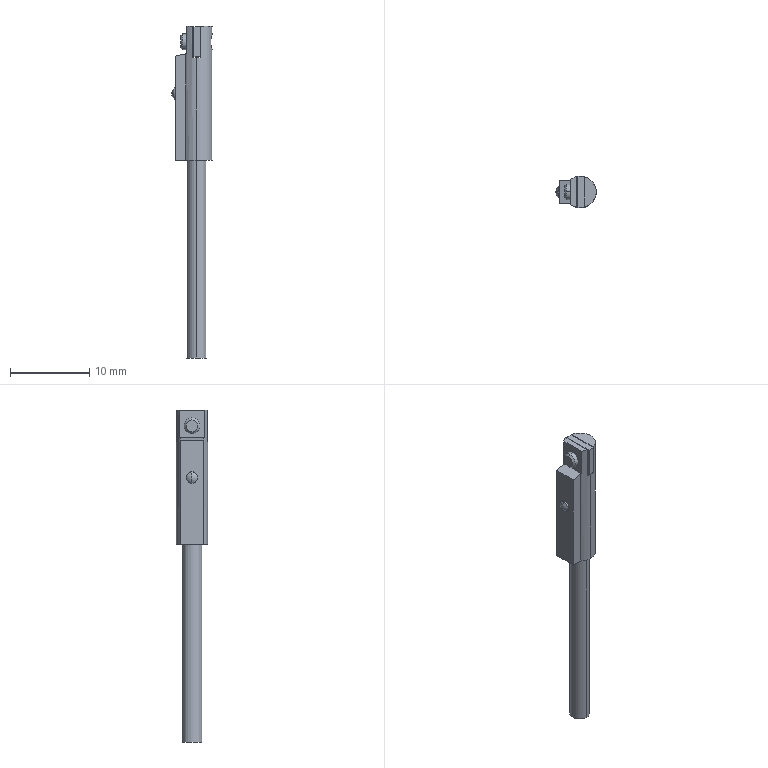Component | SolidWorks | SL010-LeftStreamline-1-1_SL010-SideClampAssembly-DB-1-1_SL010-HLQ8X10SAF(0)+(DS1-H-2)-DB-1-1_SL010-DS1-H-DB-1-1 | 1 solid | 45 faces | box 5.1 x 4 x 42 mm | volume 361 mm3 | plane 22 | cylinder 13 | cone 6 | torus 2 | sphere 2 | commonest cylinder face diameters 2 x4 4 x3 2.5 x2 1.5 x2 1.567 x2
build123d program:
from build123d import *

# Parameters (mm, degrees)
BOSS_EXTRUDE1_DEPTH      = 17
CUT_EXTRUDE1_DEPTH       = 2.5
CUT_EXTRUDE1_DEPTH_BACK  = 2.5
CUT_EXTRUDE2_DEPTH       = 4
CUT_EXTRUDE2_DEPTH_BACK  = 4
SKETCH4_W                = 4
SKETCH4_H                = 1
BOSS_EXTRUDE2_DEPTH      = 2
BOSS_EXTRUDE2_DEPTH_BACK = 2
SKETCH5_W                = 3.8
SKETCH5_H                = 0.8
SKETCH8_W                = 25
SKETCH8_H                = 1.25


with BuildPart() as part:
    # Sketch1 → Boss-Extrude1 (new body)
    with BuildSketch(Plane.XY):
        with BuildLine():
            Line((1.5, 1.323), (1.5, 2.6))
            Line((1.5, 2.6), (-1.5, 2.6))
            Line((-1.5, 2.6), (-1.5, 1.323))
            ThreePointArc((-1.5, 1.323), (0, -2), (1.5, 1.323))
        make_face()
    extrude(amount=BOSS_EXTRUDE1_DEPTH)

    # Sketch2 → Cut-Extrude1 (cut, two sides: drawn at the far end of the back side and taken through both)
    with BuildSketch(Plane(origin=(0, 0, 0), x_dir=(0, 0, -1), z_dir=(1, 0, 0)).offset(-CUT_EXTRUDE1_DEPTH_BACK)):
        Polygon((-17, 2.6), (-17, 1.22), (-13.5, 1.22), (-13.2, 2.6), align=None)
    extrude(amount=CUT_EXTRUDE1_DEPTH + CUT_EXTRUDE1_DEPTH_BACK, mode=Mode.SUBTRACT)

    # Sketch3 → Revolve1 (revolve)
    with BuildSketch(Plane(origin=(0, 0, 0), x_dir=(0, 0, -1), z_dir=(1, 0, 0)), mode=Mode.PRIVATE) as revolve1_sk:
        with BuildLine():
            Line((-7.7, 2.681), (-7.7, 2.6))
            Line((-7.7, 2.6), (-8.45, 2.6))
            Line((-8.45, 2.6), (-8.45, 3.1))
            ThreePointArc((-8.45, 3.1), (-8.08, 3.029), (-7.763, 2.826))
            ThreePointArc((-7.763, 2.826), (-7.716, 2.76), (-7.7, 2.681))
        make_face()
    revolve(revolve1_sk.sketch.rotate(Axis((0, 2.6, 8.45), (0, 1, 0)), 180), axis=Axis((0, 2.6, 8.45), (0, 1, 0)))

    # Sketch4 → Cut-Extrude2 (cut, two sides: drawn at the far end of the back side and taken through both)
    with BuildSketch(Plane(origin=(0, 0, 0), x_dir=(0, 0, -1), z_dir=(1, 0, 0)).offset(-CUT_EXTRUDE2_DEPTH_BACK)):
        with Locations((-15, 0)):
            Rectangle(SKETCH4_W, SKETCH4_H)
    extrude(amount=CUT_EXTRUDE2_DEPTH + CUT_EXTRUDE2_DEPTH_BACK, mode=Mode.SUBTRACT)

    # Sketch5 → Boss-Extrude2 (add, two sides: drawn at the far end of the back side and taken through both)
    with BuildSketch(Plane(origin=(0, 0, 0), x_dir=(0, 0, -1), z_dir=(1, 0, 0)).offset(-BOSS_EXTRUDE2_DEPTH_BACK)):
        with Locations((-15, -0.1)):
            Rectangle(SKETCH5_W, SKETCH5_H)
    extrude(amount=BOSS_EXTRUDE2_DEPTH + BOSS_EXTRUDE2_DEPTH_BACK)

    # Sketch6 → Cut-Revolve1 (revolve, cut)
    with BuildSketch(Plane(origin=(0, 0, 0), x_dir=(0, 0, -1), z_dir=(1, 0, 0)), mode=Mode.PRIVATE) as cut_revolve1_sk:
        Polygon((-15, -2), (-16, -2), (-15.784, -1.784), (-15.784, 1.103), (-16, 1.32), (-15, 1.32), align=None)
    revolve(cut_revolve1_sk.sketch.rotate(Axis((0, 1.32, 15), (0, -1, 0)), 180), axis=Axis((0, 1.32, 15), (0, -1, 0)), mode=Mode.SUBTRACT)

    # Sketch7 → Revolve2 (revolve)
    with BuildSketch(Plane(origin=(0, 0, 0), x_dir=(0, 0, -1), z_dir=(1, 0, 0)), mode=Mode.PRIVATE) as revolve2_sk:
        Polygon((-15, -1.5), (-15.755, -1.5), (-16, -1.254), (-16, 1.754), (-15.755, 2), (-15, 2), align=None)
    revolve(revolve2_sk.sketch.rotate(Axis((0, 2, 15), (0, -1, 0)), 180), axis=Axis((0, 2, 15), (0, -1, 0)))

    # Sketch8 → Revolve3 (revolve)
    with BuildSketch(Plane(origin=(0, 0, 0), x_dir=(0, 0, -1), z_dir=(1, 0, 0)), mode=Mode.PRIVATE) as revolve3_sk:
        with Locations((12.5, -0.625)):
            Rectangle(SKETCH8_W, SKETCH8_H)
    revolve(revolve3_sk.sketch.rotate(Axis((0, 0, 0), (0, 0, -1)), 90), axis=Axis((0, 0, 0), (0, 0, -1)))


solid = part.part

# Placed as in the assembly
solid = solid.moved(Location((-650.15, -112.904, -692.535), (0, 0, 90)))